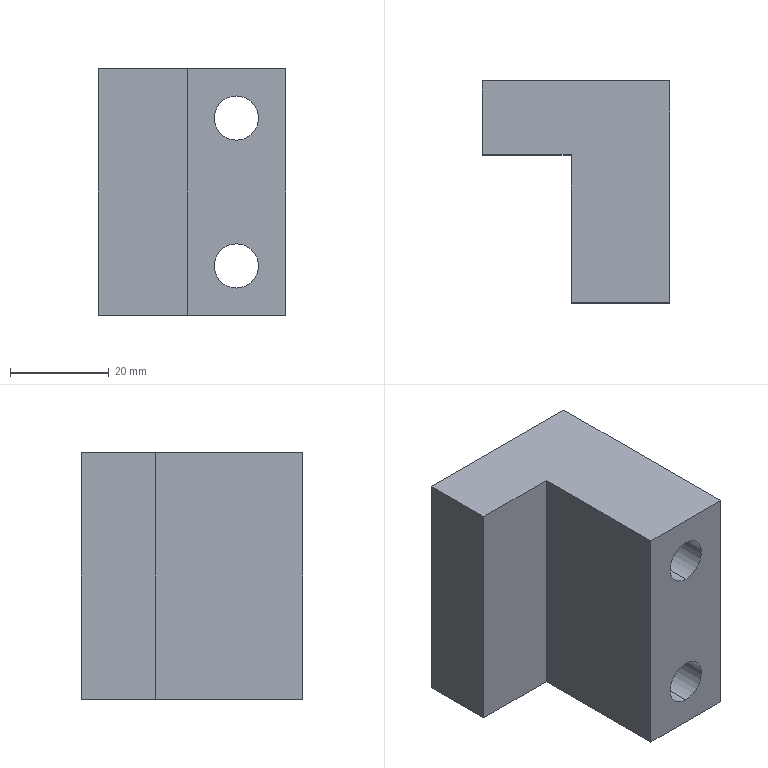Component | SolidWorks | CuttingDie-1_CuttingDieMountingSeatLocatingBlock-1 | 1 solid | 18 faces | box 38 x 45 x 50 mm | volume 51149 mm3 | plane 10 | cylinder 8 | commonest cylinder face diameters 14 x4 9 x4
build123d program:
from build123d import *

# Parameters (mm, degrees)
BOSS_EXTRUDE1_DEPTH                                 = 25
CYLINDRICAL_COUNTERSUNK_HOLE_FOR_M8_HEX_D           = 9
CYLINDRICAL_COUNTERSUNK_HOLE_FOR_M8_HEX_CBORE_D     = 14
CYLINDRICAL_COUNTERSUNK_HOLE_FOR_M8_HEX_CBORE_DEPTH = 9


with BuildPart() as part:
    # Sketch1 → Boss-Extrude1 (new, symmetric)
    with BuildSketch(Plane.XY):
        Polygon((0, 0), (38, 0), (38, -45), (18, -45), (18, -15), (0, -15), align=None)
    extrude(amount=BOSS_EXTRUDE1_DEPTH, both=True)

    # Cylindrical Countersunk Hole for M8 Hex (through all)
    with Locations(Plane(origin=(0, 0, 0), x_dir=(1, 0, 0), z_dir=(0, 1, 0))):
        with Locations((28, 15), (28, -15)):
            CounterBoreHole(CYLINDRICAL_COUNTERSUNK_HOLE_FOR_M8_HEX_D / 2, CYLINDRICAL_COUNTERSUNK_HOLE_FOR_M8_HEX_CBORE_D / 2, CYLINDRICAL_COUNTERSUNK_HOLE_FOR_M8_HEX_CBORE_DEPTH)


solid = part.part

# Placed as in the assembly
solid = solid.moved(Location((-369.772, -411.766, 1114.5), (0, 0, 0)))
STEP:
#1=COLOUR_RGB('',0.7922,0.8196,0.9333);
#2=FILL_AREA_STYLE_COLOUR('',#1);
#3=FILL_AREA_STYLE('',(#2));
#4=SURFACE_STYLE_FILL_AREA(#3);
#5=SURFACE_SIDE_STYLE('',(#4));
#6=SURFACE_STYLE_USAGE(.BOTH.,#5);
#7=PRESENTATION_STYLE_ASSIGNMENT((#6));
#8=CARTESIAN_POINT('',(-13.456,-16.566,43.012));
#9=VERTEX_POINT('',#8);
#10=CARTESIAN_POINT('',(-13.456,-16.566,43.563));
#11=VERTEX_POINT('',#10);
#12=CARTESIAN_POINT('',(-13.456,-16.566,43.287));
#13=DIRECTION('',(0.,1.,0.));
#14=DIRECTION('',(0.,0.,1.));
#15=AXIS2_PLACEMENT_3D('',#12,#13,#14);
#16=CIRCLE('',#15,0.2756);
#17=EDGE_CURVE('',#9,#11,#16,.T.);
#18=ORIENTED_EDGE('',*,*,#17,.F.);
#19=CARTESIAN_POINT('',(-13.456,-16.211,43.012));
#20=VERTEX_POINT('',#19);
#21=CARTESIAN_POINT('',(-13.456,-16.211,43.012));
#22=DIRECTION('',(0.,1.,0.));
#23=VECTOR('',#22,39.37);
#24=LINE('',#21,#23);
#25=EDGE_CURVE('',#9,#20,#24,.T.);
#26=ORIENTED_EDGE('',*,*,#25,.T.);
#27=CARTESIAN_POINT('',(-13.456,-16.211,43.563));
#28=VERTEX_POINT('',#27);
#29=CARTESIAN_POINT('',(-13.456,-16.211,43.287));
#30=DIRECTION('',(0.,1.,0.));
#31=DIRECTION('',(0.,0.,1.));
#32=AXIS2_PLACEMENT_3D('',#29,#30,#31);
#33=CIRCLE('',#32,0.2756);
#34=EDGE_CURVE('',#20,#28,#33,.T.);
#35=ORIENTED_EDGE('',*,*,#34,.T.);
#36=CARTESIAN_POINT('',(-13.456,-16.211,43.563));
#37=DIRECTION('',(0.,1.,0.));
#38=VECTOR('',#37,39.37);
#39=LINE('',#36,#38);
#40=EDGE_CURVE('',#11,#28,#39,.T.);
#41=ORIENTED_EDGE('',*,*,#40,.F.);
#42=EDGE_LOOP('',(#18,#26,#35,#41));
#43=FACE_OUTER_BOUND('',#42,.T.);
#44=CARTESIAN_POINT('',(-13.456,-16.211,43.287));
#45=DIRECTION('',(0.,1.,0.));
#46=DIRECTION('',(0.,0.,1.));
#47=AXIS2_PLACEMENT_3D('',#44,#45,#46);
#48=CYLINDRICAL_SURFACE('',#47,0.2756);
#49=ADVANCED_FACE('',(#43),#48,.F.);
#50=CARTESIAN_POINT('',(-13.456,-17.983,43.11));
#51=VERTEX_POINT('',#50);
#52=CARTESIAN_POINT('',(-13.456,-17.983,43.465));
#53=VERTEX_POINT('',#52);
#54=CARTESIAN_POINT('',(-13.456,-17.983,43.287));
#55=DIRECTION('',(0.,1.,0.));
#56=DIRECTION('',(0.,0.,1.));
#57=AXIS2_PLACEMENT_3D('',#54,#55,#56);
#58=CIRCLE('',#57,0.1772);
#59=EDGE_CURVE('',#51,#53,#58,.T.);
#60=ORIENTED_EDGE('',*,*,#59,.F.);
#61=CARTESIAN_POINT('',(-13.456,-16.566,43.11));
#62=VERTEX_POINT('',#61);
#63=CARTESIAN_POINT('',(-13.456,-16.211,43.11));
#64=DIRECTION('',(0.,1.,0.));
#65=VECTOR('',#64,39.37);
#66=LINE('',#63,#65);
#67=EDGE_CURVE('',#51,#62,#66,.T.);
#68=ORIENTED_EDGE('',*,*,#67,.T.);
#69=CARTESIAN_POINT('',(-13.456,-16.566,43.465));
#70=VERTEX_POINT('',#69);
#71=CARTESIAN_POINT('',(-13.456,-16.566,43.287));
#72=DIRECTION('',(0.,1.,0.));
#73=DIRECTION('',(0.,0.,1.));
#74=AXIS2_PLACEMENT_3D('',#71,#72,#73);
#75=CIRCLE('',#74,0.1772);
#76=EDGE_CURVE('',#62,#70,#75,.T.);
#77=ORIENTED_EDGE('',*,*,#76,.T.);
#78=CARTESIAN_POINT('',(-13.456,-16.211,43.465));
#79=DIRECTION('',(0.,1.,0.));
#80=VECTOR('',#79,39.37);
#81=LINE('',#78,#80);
#82=EDGE_CURVE('',#53,#70,#81,.T.);
#83=ORIENTED_EDGE('',*,*,#82,.F.);
#84=EDGE_LOOP('',(#60,#68,#77,#83));
#85=FACE_OUTER_BOUND('',#84,.T.);
#86=CARTESIAN_POINT('',(-13.456,-16.211,43.287));
#87=DIRECTION('',(0.,1.,0.));
#88=DIRECTION('',(0.,0.,1.));
#89=AXIS2_PLACEMENT_3D('',#86,#87,#88);
#90=CYLINDRICAL_SURFACE('',#89,0.1772);
#91=ADVANCED_FACE('',(#85),#90,.F.);
#92=CARTESIAN_POINT('',(-13.456,-16.566,44.193));
#93=VERTEX_POINT('',#92);
#94=CARTESIAN_POINT('',(-13.456,-16.566,44.744));
#95=VERTEX_POINT('',#94);
#96=CARTESIAN_POINT('',(-13.456,-16.566,44.469));
#97=DIRECTION('',(0.,1.,0.));
#98=DIRECTION('',(0.,0.,1.));
#99=AXIS2_PLACEMENT_3D('',#96,#97,#98);
#100=CIRCLE('',#99,0.2756);
#101=EDGE_CURVE('',#93,#95,#100,.T.);
#102=ORIENTED_EDGE('',*,*,#101,.F.);
#103=CARTESIAN_POINT('',(-13.456,-16.211,44.193));
#104=VERTEX_POINT('',#103);
#105=CARTESIAN_POINT('',(-13.456,-16.211,44.193));
#106=DIRECTION('',(0.,1.,0.));
#107=VECTOR('',#106,39.37);
#108=LINE('',#105,#107);
#109=EDGE_CURVE('',#93,#104,#108,.T.);
#110=ORIENTED_EDGE('',*,*,#109,.T.);
#111=CARTESIAN_POINT('',(-13.456,-16.211,44.744));
#112=VERTEX_POINT('',#111);
#113=CARTESIAN_POINT('',(-13.456,-16.211,44.469));
#114=DIRECTION('',(0.,1.,0.));
#115=DIRECTION('',(0.,0.,1.));
#116=AXIS2_PLACEMENT_3D('',#113,#114,#115);
#117=CIRCLE('',#116,0.2756);
#118=EDGE_CURVE('',#104,#112,#117,.T.);
#119=ORIENTED_EDGE('',*,*,#118,.T.);
#120=CARTESIAN_POINT('',(-13.456,-16.211,44.744));
#121=DIRECTION('',(0.,1.,0.));
#122=VECTOR('',#121,39.37);
#123=LINE('',#120,#122);
#124=EDGE_CURVE('',#95,#112,#123,.T.);
#125=ORIENTED_EDGE('',*,*,#124,.F.);
#126=EDGE_LOOP('',(#102,#110,#119,#125));
#127=FACE_OUTER_BOUND('',#126,.T.);
#128=CARTESIAN_POINT('',(-13.456,-16.211,44.469));
#129=DIRECTION('',(0.,1.,0.));
#130=DIRECTION('',(0.,0.,1.));
#131=AXIS2_PLACEMENT_3D('',#128,#129,#130);
#132=CYLINDRICAL_SURFACE('',#131,0.2756);
#133=ADVANCED_FACE('',(#127),#132,.F.);
#134=CARTESIAN_POINT('',(-13.456,-17.983,44.291));
#135=VERTEX_POINT('',#134);
#136=CARTESIAN_POINT('',(-13.456,-17.983,44.646));
#137=VERTEX_POINT('',#136);
#138=CARTESIAN_POINT('',(-13.456,-17.983,44.469));
#139=DIRECTION('',(0.,1.,0.));
#140=DIRECTION('',(0.,0.,1.));
#141=AXIS2_PLACEMENT_3D('',#138,#139,#140);
#142=CIRCLE('',#141,0.1772);
#143=EDGE_CURVE('',#135,#137,#142,.T.);
#144=ORIENTED_EDGE('',*,*,#143,.F.);
#145=CARTESIAN_POINT('',(-13.456,-16.566,44.291));
#146=VERTEX_POINT('',#145);
#147=CARTESIAN_POINT('',(-13.456,-16.211,44.291));
#148=DIRECTION('',(0.,1.,0.));
#149=VECTOR('',#148,39.37);
#150=LINE('',#147,#149);
#151=EDGE_CURVE('',#135,#146,#150,.T.);
#152=ORIENTED_EDGE('',*,*,#151,.T.);
#153=CARTESIAN_POINT('',(-13.456,-16.566,44.646));
#154=VERTEX_POINT('',#153);
#155=CARTESIAN_POINT('',(-13.456,-16.566,44.469));
#156=DIRECTION('',(0.,1.,0.));
#157=DIRECTION('',(0.,0.,1.));
#158=AXIS2_PLACEMENT_3D('',#155,#156,#157);
#159=CIRCLE('',#158,0.1772);
#160=EDGE_CURVE('',#146,#154,#159,.T.);
#161=ORIENTED_EDGE('',*,*,#160,.T.);
#162=CARTESIAN_POINT('',(-13.456,-16.211,44.646));
#163=DIRECTION('',(0.,1.,0.));
#164=VECTOR('',#163,39.37);
#165=LINE('',#162,#164);
#166=EDGE_CURVE('',#137,#154,#165,.T.);
#167=ORIENTED_EDGE('',*,*,#166,.F.);
#168=EDGE_LOOP('',(#144,#152,#161,#167));
#169=FACE_OUTER_BOUND('',#168,.T.);
#170=CARTESIAN_POINT('',(-13.456,-16.211,44.469));
#171=DIRECTION('',(0.,1.,0.));
#172=DIRECTION('',(0.,0.,1.));
#173=AXIS2_PLACEMENT_3D('',#170,#171,#172);
#174=CYLINDRICAL_SURFACE('',#173,0.1772);
#175=ADVANCED_FACE('',(#169),#174,.F.);
#176=CARTESIAN_POINT('',(-14.558,-16.211,42.894));
#177=VERTEX_POINT('',#176);
#178=CARTESIAN_POINT('',(-14.558,-16.802,42.894));
#179=VERTEX_POINT('',#178);
#180=CARTESIAN_POINT('',(-14.558,-16.802,42.894));
#181=DIRECTION('',(0.,-1.,0.));
#182=VECTOR('',#181,39.37);
#183=LINE('',#180,#182);
#184=EDGE_CURVE('',#177,#179,#183,.T.);
#185=ORIENTED_EDGE('',*,*,#184,.T.);
#186=CARTESIAN_POINT('',(-14.558,-16.802,44.862));
#187=VERTEX_POINT('',#186);
#188=CARTESIAN_POINT('',(-14.558,-16.802,44.862));
#189=DIRECTION('',(0.,0.,-1.));
#190=VECTOR('',#189,39.37);
#191=LINE('',#188,#190);
#192=EDGE_CURVE('',#187,#179,#191,.T.);
#193=ORIENTED_EDGE('',*,*,#192,.F.);
#194=CARTESIAN_POINT('',(-14.558,-16.211,44.862));
#195=VERTEX_POINT('',#194);
#196=CARTESIAN_POINT('',(-14.558,-16.802,44.862));
#197=DIRECTION('',(0.,-1.,0.));
#198=VECTOR('',#197,39.37);
#199=LINE('',#196,#198);
#200=EDGE_CURVE('',#195,#187,#199,.T.);
#201=ORIENTED_EDGE('',*,*,#200,.F.);
#202=CARTESIAN_POINT('',(-14.558,-16.211,44.862));
#203=DIRECTION('',(0.,0.,-1.));
#204=VECTOR('',#203,39.37);
#205=LINE('',#202,#204);
#206=EDGE_CURVE('',#195,#177,#205,.T.);
#207=ORIENTED_EDGE('',*,*,#206,.T.);
#208=EDGE_LOOP('',(#185,#193,#201,#207));
#209=FACE_OUTER_BOUND('',#208,.T.);
#210=CARTESIAN_POINT('',(-14.558,-16.802,44.862));
#211=DIRECTION('',(1.,0.,0.));
#212=DIRECTION('',(0.,0.,-1.));
#213=AXIS2_PLACEMENT_3D('',#210,#211,#212);
#214=PLANE('',#213);
#215=ADVANCED_FACE('',(#209),#214,.F.);
#216=CARTESIAN_POINT('',(-13.849,-16.802,42.894));
#217=VERTEX_POINT('',#216);
#218=CARTESIAN_POINT('',(-13.849,-16.802,42.894));
#219=DIRECTION('',(1.,0.,0.));
#220=VECTOR('',#219,39.37);
#221=LINE('',#218,#220);
#222=EDGE_CURVE('',#179,#217,#221,.T.);
#223=ORIENTED_EDGE('',*,*,#222,.T.);
#224=CARTESIAN_POINT('',(-13.849,-16.802,44.862));
#225=VERTEX_POINT('',#224);
#226=CARTESIAN_POINT('',(-13.849,-16.802,44.862));
#227=DIRECTION('',(0.,0.,-1.));
#228=VECTOR('',#227,39.37);
#229=LINE('',#226,#228);
#230=EDGE_CURVE('',#225,#217,#229,.T.);
#231=ORIENTED_EDGE('',*,*,#230,.F.);
#232=CARTESIAN_POINT('',(-13.849,-16.802,44.862));
#233=DIRECTION('',(1.,0.,0.));
#234=VECTOR('',#233,39.37);
#235=LINE('',#232,#234);
#236=EDGE_CURVE('',#187,#225,#235,.T.);
#237=ORIENTED_EDGE('',*,*,#236,.F.);
#238=ORIENTED_EDGE('',*,*,#192,.T.);
#239=EDGE_LOOP('',(#223,#231,#237,#238));
#240=FACE_OUTER_BOUND('',#239,.T.);
#241=CARTESIAN_POINT('',(-13.849,-16.802,44.862));
#242=DIRECTION('',(-0.,1.,0.));
#243=DIRECTION('',(-1.,-0.,0.));
#244=AXIS2_PLACEMENT_3D('',#241,#242,#243);
#245=PLANE('',#244);
#246=ADVANCED_FACE('',(#240),#245,.F.);
#247=CARTESIAN_POINT('',(-13.849,-17.983,42.894));
#248=VERTEX_POINT('',#247);
#249=CARTESIAN_POINT('',(-13.849,-17.983,42.894));
#250=DIRECTION('',(0.,-1.,0.));
#251=VECTOR('',#250,39.37);
#252=LINE('',#249,#251);
#253=EDGE_CURVE('',#217,#248,#252,.T.);
#254=ORIENTED_EDGE('',*,*,#253,.T.);
#255=CARTESIAN_POINT('',(-13.849,-17.983,44.862));
#256=VERTEX_POINT('',#255);
#257=CARTESIAN_POINT('',(-13.849,-17.983,44.862));
#258=DIRECTION('',(0.,0.,-1.));
#259=VECTOR('',#258,39.37);
#260=LINE('',#257,#259);
#261=EDGE_CURVE('',#256,#248,#260,.T.);
#262=ORIENTED_EDGE('',*,*,#261,.F.);
#263=CARTESIAN_POINT('',(-13.849,-17.983,44.862));
#264=DIRECTION('',(0.,-1.,0.));
#265=VECTOR('',#264,39.37);
#266=LINE('',#263,#265);
#267=EDGE_CURVE('',#225,#256,#266,.T.);
#268=ORIENTED_EDGE('',*,*,#267,.F.);
#269=ORIENTED_EDGE('',*,*,#230,.T.);
#270=EDGE_LOOP('',(#254,#262,#268,#269));
#271=FACE_OUTER_BOUND('',#270,.T.);
#272=CARTESIAN_POINT('',(-13.849,-17.983,44.862));
#273=DIRECTION('',(1.,0.,0.));
#274=DIRECTION('',(-0.,1.,0.));
#275=AXIS2_PLACEMENT_3D('',#272,#273,#274);
#276=PLANE('',#275);
#277=ADVANCED_FACE('',(#271),#276,.F.);
#278=CARTESIAN_POINT('',(-13.456,-17.983,43.287));
#279=DIRECTION('',(0.,1.,0.));
#280=DIRECTION('',(0.,0.,1.));
#281=AXIS2_PLACEMENT_3D('',#278,#279,#280);
#282=CIRCLE('',#281,0.1772);
#283=EDGE_CURVE('',#53,#51,#282,.T.);
#284=ORIENTED_EDGE('',*,*,#283,.T.);
#285=ORIENTED_EDGE('',*,*,#59,.T.);
#286=EDGE_LOOP('',(#284,#285));
#287=FACE_BOUND('',#286,.T.);
#288=CARTESIAN_POINT('',(-13.456,-17.983,44.469));
#289=DIRECTION('',(0.,1.,0.));
#290=DIRECTION('',(0.,0.,1.));
#291=AXIS2_PLACEMENT_3D('',#288,#289,#290);
#292=CIRCLE('',#291,0.1772);
#293=EDGE_CURVE('',#137,#135,#292,.T.);
#294=ORIENTED_EDGE('',*,*,#293,.T.);
#295=ORIENTED_EDGE('',*,*,#143,.T.);
#296=EDGE_LOOP('',(#294,#295));
#297=FACE_BOUND('',#296,.T.);
#298=CARTESIAN_POINT('',(-13.062,-17.983,42.894));
#299=VERTEX_POINT('',#298);
#300=CARTESIAN_POINT('',(-13.062,-17.983,42.894));
#301=DIRECTION('',(1.,0.,0.));
#302=VECTOR('',#301,39.37);
#303=LINE('',#300,#302);
#304=EDGE_CURVE('',#248,#299,#303,.T.);
#305=ORIENTED_EDGE('',*,*,#304,.T.);
#306=CARTESIAN_POINT('',(-13.062,-17.983,44.862));
#307=VERTEX_POINT('',#306);
#308=CARTESIAN_POINT('',(-13.062,-17.983,44.862));
#309=DIRECTION('',(0.,0.,-1.));
#310=VECTOR('',#309,39.37);
#311=LINE('',#308,#310);
#312=EDGE_CURVE('',#307,#299,#311,.T.);
#313=ORIENTED_EDGE('',*,*,#312,.F.);
#314=CARTESIAN_POINT('',(-13.062,-17.983,44.862));
#315=DIRECTION('',(1.,0.,0.));
#316=VECTOR('',#315,39.37);
#317=LINE('',#314,#316);
#318=EDGE_CURVE('',#256,#307,#317,.T.);
#319=ORIENTED_EDGE('',*,*,#318,.F.);
#320=ORIENTED_EDGE('',*,*,#261,.T.);
#321=EDGE_LOOP('',(#305,#313,#319,#320));
#322=FACE_OUTER_BOUND('',#321,.T.);
#323=CARTESIAN_POINT('',(-13.062,-17.983,44.862));
#324=DIRECTION('',(0.,1.,0.));
#325=DIRECTION('',(0.,0.,1.));
#326=AXIS2_PLACEMENT_3D('',#323,#324,#325);
#327=PLANE('',#326);
#328=ADVANCED_FACE('',(#287,#297,#322),#327,.F.);
#329=CARTESIAN_POINT('',(-13.062,-16.211,42.894));
#330=VERTEX_POINT('',#329);
#331=CARTESIAN_POINT('',(-13.062,-16.211,42.894));
#332=DIRECTION('',(-0.,1.,0.));
#333=VECTOR('',#332,39.37);
#334=LINE('',#331,#333);
#335=EDGE_CURVE('',#299,#330,#334,.T.);
#336=ORIENTED_EDGE('',*,*,#335,.T.);
#337=CARTESIAN_POINT('',(-13.062,-16.211,44.862));
#338=VERTEX_POINT('',#337);
#339=CARTESIAN_POINT('',(-13.062,-16.211,44.862));
#340=DIRECTION('',(0.,0.,-1.));
#341=VECTOR('',#340,39.37);
#342=LINE('',#339,#341);
#343=EDGE_CURVE('',#338,#330,#342,.T.);
#344=ORIENTED_EDGE('',*,*,#343,.F.);
#345=CARTESIAN_POINT('',(-13.062,-16.211,44.862));
#346=DIRECTION('',(-0.,1.,0.));
#347=VECTOR('',#346,39.37);
#348=LINE('',#345,#347);
#349=EDGE_CURVE('',#307,#338,#348,.T.);
#350=ORIENTED_EDGE('',*,*,#349,.F.);
#351=ORIENTED_EDGE('',*,*,#312,.T.);
#352=EDGE_LOOP('',(#336,#344,#350,#351));
#353=FACE_OUTER_BOUND('',#352,.T.);
#354=CARTESIAN_POINT('',(-13.062,-16.211,44.862));
#355=DIRECTION('',(-1.,-0.,0.));
#356=DIRECTION('',(0.,-1.,0.));
#357=AXIS2_PLACEMENT_3D('',#354,#355,#356);
#358=PLANE('',#357);
#359=ADVANCED_FACE('',(#353),#358,.F.);
#360=CARTESIAN_POINT('',(-13.456,-16.211,43.287));
#361=DIRECTION('',(0.,1.,0.));
#362=DIRECTION('',(0.,0.,1.));
#363=AXIS2_PLACEMENT_3D('',#360,#361,#362);
#364=CIRCLE('',#363,0.2756);
#365=EDGE_CURVE('',#28,#20,#364,.T.);
#366=ORIENTED_EDGE('',*,*,#365,.F.);
#367=ORIENTED_EDGE('',*,*,#34,.F.);
#368=EDGE_LOOP('',(#366,#367));
#369=FACE_BOUND('',#368,.T.);
#370=CARTESIAN_POINT('',(-13.456,-16.211,44.469));
#371=DIRECTION('',(0.,1.,0.));
#372=DIRECTION('',(0.,0.,1.));
#373=AXIS2_PLACEMENT_3D('',#370,#371,#372);
#374=CIRCLE('',#373,0.2756);
#375=EDGE_CURVE('',#112,#104,#374,.T.);
#376=ORIENTED_EDGE('',*,*,#375,.F.);
#377=ORIENTED_EDGE('',*,*,#118,.F.);
#378=EDGE_LOOP('',(#376,#377));
#379=FACE_BOUND('',#378,.T.);
#380=CARTESIAN_POINT('',(-14.558,-16.211,42.894));
#381=DIRECTION('',(-1.,0.,0.));
#382=VECTOR('',#381,39.37);
#383=LINE('',#380,#382);
#384=EDGE_CURVE('',#330,#177,#383,.T.);
#385=ORIENTED_EDGE('',*,*,#384,.T.);
#386=ORIENTED_EDGE('',*,*,#206,.F.);
#387=CARTESIAN_POINT('',(-14.558,-16.211,44.862));
#388=DIRECTION('',(-1.,0.,0.));
#389=VECTOR('',#388,39.37);
#390=LINE('',#387,#389);
#391=EDGE_CURVE('',#338,#195,#390,.T.);
#392=ORIENTED_EDGE('',*,*,#391,.F.);
#393=ORIENTED_EDGE('',*,*,#343,.T.);
#394=EDGE_LOOP('',(#385,#386,#392,#393));
#395=FACE_OUTER_BOUND('',#394,.T.);
#396=CARTESIAN_POINT('',(-14.558,-16.211,44.862));
#397=DIRECTION('',(0.,-1.,0.));
#398=DIRECTION('',(0.,0.,-1.));
#399=AXIS2_PLACEMENT_3D('',#396,#397,#398);
#400=PLANE('',#399);
#401=ADVANCED_FACE('',(#369,#379,#395),#400,.F.);
#402=ORIENTED_EDGE('',*,*,#200,.T.);
#403=ORIENTED_EDGE('',*,*,#236,.T.);
#404=ORIENTED_EDGE('',*,*,#267,.T.);
#405=ORIENTED_EDGE('',*,*,#318,.T.);
#406=ORIENTED_EDGE('',*,*,#349,.T.);
#407=ORIENTED_EDGE('',*,*,#391,.T.);
#408=EDGE_LOOP('',(#402,#403,#404,#405,#406,#407));
#409=FACE_OUTER_BOUND('',#408,.T.);
#410=CARTESIAN_POINT('',(-14.558,-16.211,44.862));
#411=DIRECTION('',(0.,0.,-1.));
#412=DIRECTION('',(-1.,0.,0.));
#413=AXIS2_PLACEMENT_3D('',#410,#411,#412);
#414=PLANE('',#413);
#415=ADVANCED_FACE('',(#409),#414,.F.);
#416=ORIENTED_EDGE('',*,*,#184,.F.);
#417=ORIENTED_EDGE('',*,*,#384,.F.);
#418=ORIENTED_EDGE('',*,*,#335,.F.);
#419=ORIENTED_EDGE('',*,*,#304,.F.);
#420=ORIENTED_EDGE('',*,*,#253,.F.);
#421=ORIENTED_EDGE('',*,*,#222,.F.);
#422=EDGE_LOOP('',(#416,#417,#418,#419,#420,#421));
#423=FACE_OUTER_BOUND('',#422,.T.);
#424=CARTESIAN_POINT('',(-14.558,-16.211,42.894));
#425=DIRECTION('',(0.,0.,-1.));
#426=DIRECTION('',(-1.,0.,0.));
#427=AXIS2_PLACEMENT_3D('',#424,#425,#426);
#428=PLANE('',#427);
#429=ADVANCED_FACE('',(#423),#428,.T.);
#430=ORIENTED_EDGE('',*,*,#151,.F.);
#431=ORIENTED_EDGE('',*,*,#293,.F.);
#432=ORIENTED_EDGE('',*,*,#166,.T.);
#433=CARTESIAN_POINT('',(-13.456,-16.566,44.469));
#434=DIRECTION('',(0.,1.,0.));
#435=DIRECTION('',(0.,0.,1.));
#436=AXIS2_PLACEMENT_3D('',#433,#434,#435);
#437=CIRCLE('',#436,0.1772);
#438=EDGE_CURVE('',#154,#146,#437,.T.);
#439=ORIENTED_EDGE('',*,*,#438,.T.);
#440=EDGE_LOOP('',(#430,#431,#432,#439));
#441=FACE_OUTER_BOUND('',#440,.T.);
#442=CARTESIAN_POINT('',(-13.456,-16.211,44.469));
#443=DIRECTION('',(0.,1.,0.));
#444=DIRECTION('',(0.,0.,1.));
#445=AXIS2_PLACEMENT_3D('',#442,#443,#444);
#446=CYLINDRICAL_SURFACE('',#445,0.1772);
#447=ADVANCED_FACE('',(#441),#446,.F.);
#448=ORIENTED_EDGE('',*,*,#438,.F.);
#449=ORIENTED_EDGE('',*,*,#160,.F.);
#450=EDGE_LOOP('',(#448,#449));
#451=FACE_BOUND('',#450,.T.);
#452=CARTESIAN_POINT('',(-13.456,-16.566,44.469));
#453=DIRECTION('',(0.,1.,0.));
#454=DIRECTION('',(0.,0.,1.));
#455=AXIS2_PLACEMENT_3D('',#452,#453,#454);
#456=CIRCLE('',#455,0.2756);
#457=EDGE_CURVE('',#95,#93,#456,.T.);
#458=ORIENTED_EDGE('',*,*,#457,.T.);
#459=ORIENTED_EDGE('',*,*,#101,.T.);
#460=EDGE_LOOP('',(#458,#459));
#461=FACE_OUTER_BOUND('',#460,.T.);
#462=CARTESIAN_POINT('',(-13.278,-16.566,44.469));
#463=DIRECTION('',(0.,-1.,0.));
#464=DIRECTION('',(0.,0.,-1.));
#465=AXIS2_PLACEMENT_3D('',#462,#463,#464);
#466=PLANE('',#465);
#467=ADVANCED_FACE('',(#451,#461),#466,.F.);
#468=ORIENTED_EDGE('',*,*,#109,.F.);
#469=ORIENTED_EDGE('',*,*,#457,.F.);
#470=ORIENTED_EDGE('',*,*,#124,.T.);
#471=ORIENTED_EDGE('',*,*,#375,.T.);
#472=EDGE_LOOP('',(#468,#469,#470,#471));
#473=FACE_OUTER_BOUND('',#472,.T.);
#474=CARTESIAN_POINT('',(-13.456,-16.211,44.469));
#475=DIRECTION('',(0.,1.,0.));
#476=DIRECTION('',(0.,0.,1.));
#477=AXIS2_PLACEMENT_3D('',#474,#475,#476);
#478=CYLINDRICAL_SURFACE('',#477,0.2756);
#479=ADVANCED_FACE('',(#473),#478,.F.);
#480=ORIENTED_EDGE('',*,*,#67,.F.);
#481=ORIENTED_EDGE('',*,*,#283,.F.);
#482=ORIENTED_EDGE('',*,*,#82,.T.);
#483=CARTESIAN_POINT('',(-13.456,-16.566,43.287));
#484=DIRECTION('',(0.,1.,0.));
#485=DIRECTION('',(0.,0.,1.));
#486=AXIS2_PLACEMENT_3D('',#483,#484,#485);
#487=CIRCLE('',#486,0.1772);
#488=EDGE_CURVE('',#70,#62,#487,.T.);
#489=ORIENTED_EDGE('',*,*,#488,.T.);
#490=EDGE_LOOP('',(#480,#481,#482,#489));
#491=FACE_OUTER_BOUND('',#490,.T.);
#492=CARTESIAN_POINT('',(-13.456,-16.211,43.287));
#493=DIRECTION('',(0.,1.,0.));
#494=DIRECTION('',(0.,0.,1.));
#495=AXIS2_PLACEMENT_3D('',#492,#493,#494);
#496=CYLINDRICAL_SURFACE('',#495,0.1772);
#497=ADVANCED_FACE('',(#491),#496,.F.);
#498=ORIENTED_EDGE('',*,*,#488,.F.);
#499=ORIENTED_EDGE('',*,*,#76,.F.);
#500=EDGE_LOOP('',(#498,#499));
#501=FACE_BOUND('',#500,.T.);
#502=CARTESIAN_POINT('',(-13.456,-16.566,43.287));
#503=DIRECTION('',(0.,1.,0.));
#504=DIRECTION('',(0.,0.,1.));
#505=AXIS2_PLACEMENT_3D('',#502,#503,#504);
#506=CIRCLE('',#505,0.2756);
#507=EDGE_CURVE('',#11,#9,#506,.T.);
#508=ORIENTED_EDGE('',*,*,#507,.T.);
#509=ORIENTED_EDGE('',*,*,#17,.T.);
#510=EDGE_LOOP('',(#508,#509));
#511=FACE_OUTER_BOUND('',#510,.T.);
#512=CARTESIAN_POINT('',(-13.278,-16.566,43.287));
#513=DIRECTION('',(0.,-1.,0.));
#514=DIRECTION('',(0.,0.,-1.));
#515=AXIS2_PLACEMENT_3D('',#512,#513,#514);
#516=PLANE('',#515);
#517=ADVANCED_FACE('',(#501,#511),#516,.F.);
#518=ORIENTED_EDGE('',*,*,#25,.F.);
#519=ORIENTED_EDGE('',*,*,#507,.F.);
#520=ORIENTED_EDGE('',*,*,#40,.T.);
#521=ORIENTED_EDGE('',*,*,#365,.T.);
#522=EDGE_LOOP('',(#518,#519,#520,#521));
#523=FACE_OUTER_BOUND('',#522,.T.);
#524=CARTESIAN_POINT('',(-13.456,-16.211,43.287));
#525=DIRECTION('',(0.,1.,0.));
#526=DIRECTION('',(0.,0.,1.));
#527=AXIS2_PLACEMENT_3D('',#524,#525,#526);
#528=CYLINDRICAL_SURFACE('',#527,0.2756);
#529=ADVANCED_FACE('',(#523),#528,.F.);
#530=CLOSED_SHELL('',(#49,#91,#133,#175,#215,#246,#277,#328,#359,#401,#415,#429,#447,#467,#479,#497,#517,#529));
#531=MANIFOLD_SOLID_BREP('',#530);
#532=STYLED_ITEM('',(#7),#531);
#533=PRESENTATION_LAYER_ASSIGNMENT('','',(#532));
#534=CARTESIAN_POINT('',(0.,0.,0.));
#535=DIRECTION('',(0.,0.,1.));
#536=DIRECTION('',(1.,0.,0.));
#537=AXIS2_PLACEMENT_3D('',#534,#535,#536);
#538=(LENGTH_UNIT()NAMED_UNIT(*)SI_UNIT($,.METRE.));
#539=LENGTH_MEASURE_WITH_UNIT(LENGTH_MEASURE(0.0254),#538);
#540=DIMENSIONAL_EXPONENTS(1.,0.,0.,0.,0.,0.,0.);
#541=(CONVERSION_BASED_UNIT('',#539)LENGTH_UNIT()NAMED_UNIT(#540));
#542=UNCERTAINTY_MEASURE_WITH_UNIT(LENGTH_MEASURE(0.00001),#541,'','');
#543=(NAMED_UNIT(*)PLANE_ANGLE_UNIT()SI_UNIT($,.RADIAN.));
#544=(NAMED_UNIT(*)SI_UNIT($,.STERADIAN.)SOLID_ANGLE_UNIT());
#545=(GEOMETRIC_REPRESENTATION_CONTEXT(3)GLOBAL_UNCERTAINTY_ASSIGNED_CONTEXT((#542))GLOBAL_UNIT_ASSIGNED_CONTEXT((#541,#543,#544))REPRESENTATION_CONTEXT('',''));
#546=ADVANCED_BREP_SHAPE_REPRESENTATION('',(#531,#537),#545);
#547=(LENGTH_UNIT()NAMED_UNIT(*)SI_UNIT($,.METRE.));
#548=LENGTH_MEASURE_WITH_UNIT(LENGTH_MEASURE(0.0254),#547);
#549=DIMENSIONAL_EXPONENTS(1.,0.,0.,0.,0.,0.,0.);
#550=(CONVERSION_BASED_UNIT('',#548)LENGTH_UNIT()NAMED_UNIT(#549));
#551=UNCERTAINTY_MEASURE_WITH_UNIT(LENGTH_MEASURE(0.00001),#550,'','');
#552=(NAMED_UNIT(*)PLANE_ANGLE_UNIT()SI_UNIT($,.RADIAN.));
#553=(NAMED_UNIT(*)SI_UNIT($,.STERADIAN.)SOLID_ANGLE_UNIT());
#554=(GEOMETRIC_REPRESENTATION_CONTEXT(3)GLOBAL_UNCERTAINTY_ASSIGNED_CONTEXT((#551))GLOBAL_UNIT_ASSIGNED_CONTEXT((#550,#552,#553))REPRESENTATION_CONTEXT('',''));
#555=MECHANICAL_DESIGN_GEOMETRIC_PRESENTATION_REPRESENTATION('',(#532),#554);